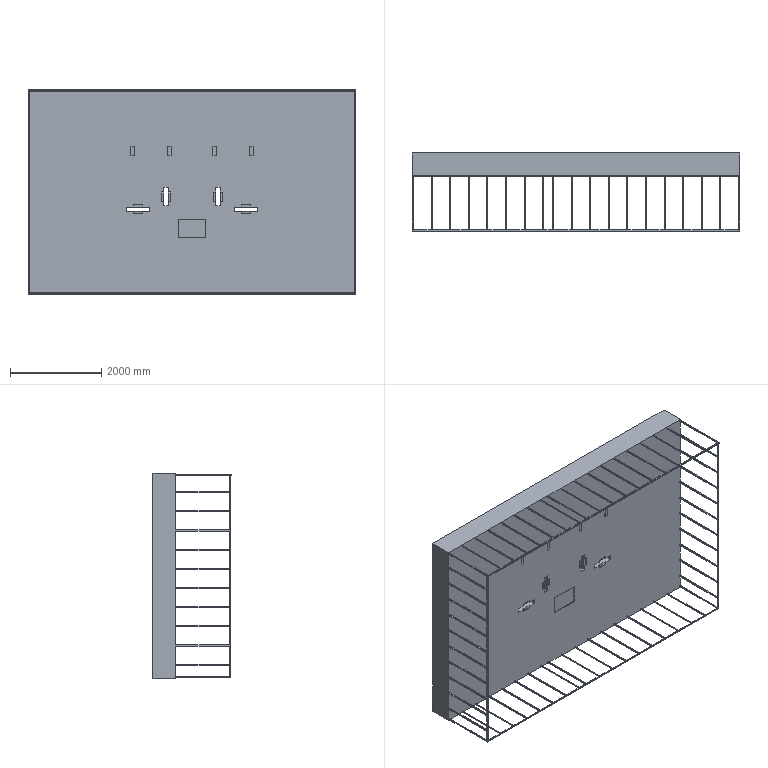Component | SolidWorks | LiftingAndOperatingMechanism-1_16-1 | 1 solid | 261 faces | box 7170 x 1712.5 x 4500 mm | volume 16079482000 mm3 | plane 261
build123d program:
from build123d import *

# Parameters (mm, degrees)
SKETCH1_W            = 4500
SKETCH1_H            = 7170
BOSS_EXTRUDE1_DEPTH  = 500
SKETCH6_W            = 20
SKETCH6_H            = 20
BOSS_EXTRUDE5_DEPTH  = 1200
SKETCH7_W            = 20
SKETCH7_H            = 7170
BOSS_EXTRUDE6_DEPTH  = 20
SKETCH9_W            = 100
SKETCH9_H            = 500
SKETCH9_W_2          = 400
SKETCH9_H_2          = 100
CUT_EXTRUDE2_DEPTH   = 4400.401
SKETCH10_W           = 400
SKETCH10_H           = 600
CUT_EXTRUDE3_DEPTH   = 20
SKETCH15_W           = 200
SKETCH15_H           = 200
CUT_EXTRUDE4_DEPTH   = 20
SKETCH16_W           = 200
SKETCH16_H           = 80
CUT_EXTRUDE5_DEPTH   = 20
SKETCH17_W           = 20
SKETCH17_H           = 7170
BOSS_EXTRUDE7_DEPTH  = 12.5
SKETCH19_W           = 25
SKETCH19_H           = 25
BOSS_EXTRUDE9_DEPTH  = 1200
SKETCH20_W           = 4460
SKETCH20_H           = 25
BOSS_EXTRUDE12_DEPTH = 25


with BuildPart() as part:
    # Sketch1 → Boss-Extrude1 (new body)
    with BuildSketch(Plane(origin=(0, 0, 0), x_dir=(1, 0, 0), z_dir=(0, 1, 0))):
        Rectangle(SKETCH1_W, SKETCH1_H)
    extrude(amount=BOSS_EXTRUDE1_DEPTH)

    # Sketch6 → Boss-Extrude5 (add)
    with BuildSketch(Plane(origin=(0, 500, 0), x_dir=(1, 0, 0), z_dir=(0, 1, 0))):
        with Locations((2220, 3575)):
            Rectangle(SKETCH6_W, SKETCH6_H)
        with Locations((2220, 3167)):
            Rectangle(SKETCH6_W, SKETCH6_H)
        with Locations((2220, 2759)):
            Rectangle(SKETCH6_W, SKETCH6_H)
        with Locations((2220, 2351)):
            Rectangle(SKETCH6_W, SKETCH6_H)
        with Locations((2220, 1943)):
            Rectangle(SKETCH6_W, SKETCH6_H)
        with Locations((2220, 1535)):
            Rectangle(SKETCH6_W, SKETCH6_H)
        with Locations((2220, 1127)):
            Rectangle(SKETCH6_W, SKETCH6_H)
        with Locations((2220, 719)):
            Rectangle(SKETCH6_W, SKETCH6_H)
        with Locations((2220, -719)):
            Rectangle(SKETCH6_W, SKETCH6_H)
        with Locations((2220, -1127)):
            Rectangle(SKETCH6_W, SKETCH6_H)
        with Locations((2220, -1535)):
            Rectangle(SKETCH6_W, SKETCH6_H)
        with Locations((2220, -1943)):
            Rectangle(SKETCH6_W, SKETCH6_H)
        with Locations((2220, -2351)):
            Rectangle(SKETCH6_W, SKETCH6_H)
        with Locations((2220, -2759)):
            Rectangle(SKETCH6_W, SKETCH6_H)
        with Locations((2220, -3167)):
            Rectangle(SKETCH6_W, SKETCH6_H)
        with Locations((2220, -3575)):
            Rectangle(SKETCH6_W, SKETCH6_H)
        with Locations((2220, 311)):
            Rectangle(SKETCH6_W, SKETCH6_H)
        with Locations((2220, -97)):
            Rectangle(SKETCH6_W, SKETCH6_H)
        with Locations((2220, -505)):
            Rectangle(SKETCH6_W, SKETCH6_H)
    boss_extrude5 = extrude(amount=BOSS_EXTRUDE5_DEPTH)

    # Sketch7 → Boss-Extrude6 (add)
    with BuildSketch(Plane(origin=(0, 1700, 0), x_dir=(1, 0, 0), z_dir=(0, 1, 0))):
        with Locations((2220, 0)):
            Rectangle(SKETCH7_W, SKETCH7_H)
    extrude(amount=-BOSS_EXTRUDE6_DEPTH)

    # Sketch9 → Cut-Extrude2 (cut, through all)
    with BuildSketch(Plane(origin=(0, 500, 0), x_dir=(1, 0, 0), z_dir=(0, 1, 0))):
        with Locations((380, 1180)):
            Rectangle(SKETCH9_W, SKETCH9_H)
        with Locations((100, 570)):
            Rectangle(SKETCH9_W_2, SKETCH9_H_2)
        with Locations((100, -570)):
            Rectangle(SKETCH9_W_2, SKETCH9_H_2)
        with Locations((380, -1180)):
            Rectangle(SKETCH9_W, SKETCH9_H)
    extrude(amount=-CUT_EXTRUDE2_DEPTH, mode=Mode.SUBTRACT)

    # Sketch10 → Cut-Extrude3 (cut)
    with BuildSketch(Plane(origin=(0, 500, 0), x_dir=(1, 0, 0), z_dir=(0, 1, 0))):
        with Locations((800, 0)):
            Rectangle(SKETCH10_W, SKETCH10_H)
    extrude(amount=-CUT_EXTRUDE3_DEPTH, mode=Mode.SUBTRACT)

    # Sketch15 → Cut-Extrude4 (cut)
    with BuildSketch(Plane(origin=(0, 500, 0), x_dir=(1, 0, 0), z_dir=(0, 1, 0))):
        with Locations((380, 1180)):
            Rectangle(SKETCH15_W, SKETCH15_H)
        with Locations((100, 570)):
            Rectangle(SKETCH15_W, SKETCH15_H)
        with Locations((100, -570)):
            Rectangle(SKETCH15_W, SKETCH15_H)
        with Locations((380, -1180)):
            Rectangle(SKETCH15_W, SKETCH15_H)
    extrude(amount=-CUT_EXTRUDE4_DEPTH, mode=Mode.SUBTRACT)

    # Sketch16 → Cut-Extrude5 (cut)
    with BuildSketch(Plane(origin=(0, 500, 0), x_dir=(1, 0, 0), z_dir=(0, 1, 0))):
        with Locations((-900, 1300)):
            Rectangle(SKETCH16_W, SKETCH16_H)
        with Locations((-900, 500)):
            Rectangle(SKETCH16_W, SKETCH16_H)
        with Locations((-900, -500)):
            Rectangle(SKETCH16_W, SKETCH16_H)
        with Locations((-900, -1300)):
            Rectangle(SKETCH16_W, SKETCH16_H)
    extrude(amount=-CUT_EXTRUDE5_DEPTH, mode=Mode.SUBTRACT)

    # Mirror1: Boss-Extrude5 across plane
    add(boss_extrude5.mirror(Plane(origin=(0, 0, 0), x_dir=(0, 0, 1), z_dir=(1, 0, 0))))

    # Sketch17 → Boss-Extrude7 (add, symmetric)
    with BuildSketch(Plane(origin=(0, 1700, 0), x_dir=(1, 0, 0), z_dir=(0, 1, 0))):
        with Locations((-2220, 0)):
            Rectangle(SKETCH17_W, SKETCH17_H)
    extrude(amount=BOSS_EXTRUDE7_DEPTH, both=True)

    # Sketch19 → Boss-Extrude9 (add)
    with BuildSketch(Plane(origin=(0, 500, 0), x_dir=(1, 0, 0), z_dir=(0, 1, 0))):
        with Locations((-1837.5, 3572.5)):
            Rectangle(SKETCH19_W, SKETCH19_H)
        with Locations((-1417.5, 3572.5)):
            Rectangle(SKETCH19_W, SKETCH19_H)
        with Locations((-997.5, 3572.5)):
            Rectangle(SKETCH19_W, SKETCH19_H)
        with Locations((-577.5, 3572.5)):
            Rectangle(SKETCH19_W, SKETCH19_H)
        with Locations((-157.5, 3572.5)):
            Rectangle(SKETCH19_W, SKETCH19_H)
        with Locations((262.5, 3572.5)):
            Rectangle(SKETCH19_W, SKETCH19_H)
        with Locations((682.5, 3572.5)):
            Rectangle(SKETCH19_W, SKETCH19_H)
        with Locations((1102.5, 3572.5)):
            Rectangle(SKETCH19_W, SKETCH19_H)
        with Locations((1522.5, 3572.5)):
            Rectangle(SKETCH19_W, SKETCH19_H)
        with Locations((1942.5, 3572.5)):
            Rectangle(SKETCH19_W, SKETCH19_H)
    boss_extrude9 = extrude(amount=BOSS_EXTRUDE9_DEPTH)

    # Sketch20 → Boss-Extrude12 (add)
    with BuildSketch(Plane(origin=(0, 1700, 0), x_dir=(1, 0, 0), z_dir=(0, 1, 0))):
        with Locations((0, 3572.5)):
            Rectangle(SKETCH20_W, SKETCH20_H)
    boss_extrude12 = extrude(amount=-BOSS_EXTRUDE12_DEPTH)

    # Mirror2: Boss-Extrude9, Boss-Extrude12 across plane
    add(boss_extrude9.mirror(Plane.XY))
    add(boss_extrude12.mirror(Plane.XY))


solid = part.part

# Placed as in the assembly
solid = solid.moved(Location((-258.963, 12918.918, 6632.153), (180, -90, 0)))